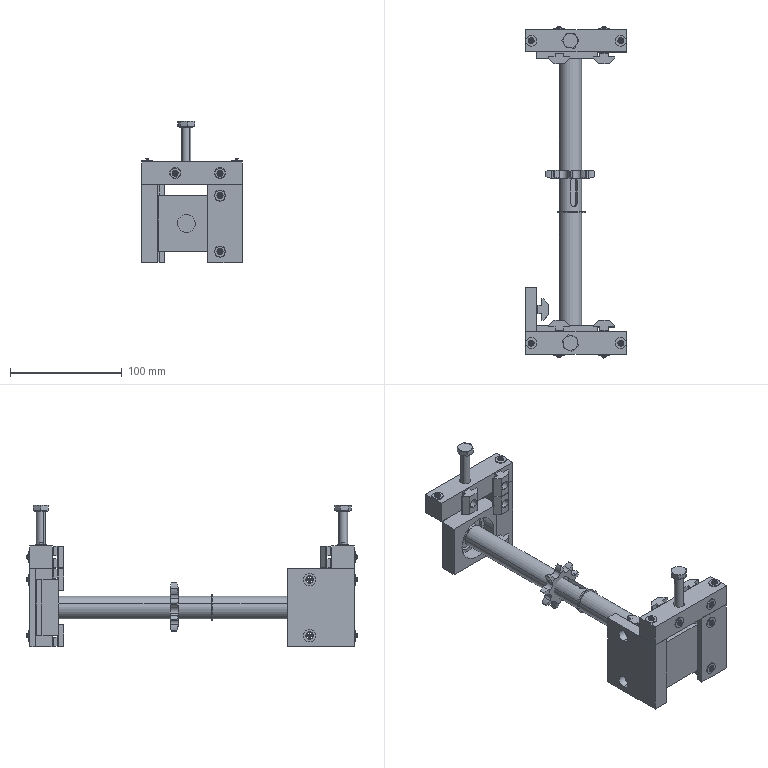Assembly | SolidWorks | mm | 63 component files | 63 solids | 1262 faces | box 90 x 296.4 x 126.4 mm | volume 353563 mm3 | plane 541 | cylinder 367 | torus 158 | sphere 100 | cone 96 | commonest cylinder face diameters 3 x64 4.2 x36 10 x28 1.6 x28 5.5 x24 6 x23 8 x20 22.466 x19
Bill of materials:
CTM-T-12-AG-02 | 2 | Q235A | Long rectangular bar with three through holes in the top face (a larger one near the middle and a smaller one near each end) and two cross holes through one long side face.
CTM-T-12-AG-03 | 1 | Q235A | Thick rectangular plate with an L-shaped profile: a small step or lip runs along one edge. Two through holes pass through the large face, and one hole is drilled into the narrow top end face.
CTM-T-12-AG-04 | 2 | Q235A | Solid rectangular block with a stepped (tongue-like) profile: a narrower raised section projects from one face, and a small notch shows at one top corner in isometric. No holes visible.
CTM-T-12-AG-05 | 2 | Q235A | Upright rectangular block with a rectangular notch (rabbet) at one top corner. Two through holes pass through one side face, and a single hole is drilled into the top face.
CTM-T-12-D-GD-03 | 1 | 45 | Stepped cylindrical shaft or pin: reduced-diameter journals at both ends and a slot (keyway-like) on the central section. Several circumferential seam lines divide the body into segments.
hex head bolts-full thread grade c gb | 2 |  | Hex-head bolt shape: chamfered hexagonal head on a plain cylindrical shank with a chamfered tip.
hexagon socket head cap screws gb | 14 |  | Socket-head cap screw shape: cylindrical head with a hexagonal socket recess, a plain cylindrical shank, and a chamfered end.
plain washers--product grade c gb | 12 |  | Plain flat washer: a thin annular disc with a central round hole.
self-aligning ball bearings gb | 2 |  | Ball-bearing-like assembly: an outer ring and an inner ring with a single row of 12 visible spherical rolling elements between them. No cage or shields visible.
ShaftRetainingRingTypeA-20-GB894.1-1986 | 2 | 65Mn | Flat split retaining ring (circlip shape) with a gap and two lugs, each with a small hole, beside the opening.
short pitch roller chain wheel_s_iso | 1 |  | Toothed disc with 9 teeth, rounded tooth gaps, and a plain central round bore; resembles a small chain sprocket.
spring lock washers--normal type gb | 12 |  | Split ring with a rectangular cross-section and one angled cut through the ring; resembles a split lock washer.
SquareNutBlock-MC6-8-30 | 2 | Purchased Part | Prismatic block with a constant T-shaped cross-section: a narrow rectangular stem on one side of a wider head whose outer edges are chamfered at about 45 degrees. One round through-hole runs through the wide flat face, roughly centred.
SquareNutBlock-MC8-8-40 | 8 | Purchased Part | Prismatic block with a T-shaped cross-section: a rectangular stem under a wider head with chamfered sides. A large round through-hole runs through the square face. A narrow rectangular slot is cut across the stem, partway into its depth, and meets the hole.
Mates:
1. concentric | self-aligning ball bearings gb-2 face at (40.4, -17, 35) dir (0, 1, 0) r 3 | CTM-T-12-D-GD-03-1 face at (40.4, -7, 35) dir (0, -1, 0) r 8.5
2. concentric | CTM-T-12-D-GD-03-1 face at (40.4, -270, 35) dir (0, 1, 0) r 10 | short pitch roller chain wheel_s_iso-1 face at (40.4, -123.269, 35) dir (0, -1, 0) r 6
3. width | self-aligning ball bearings gb-2 face at (43.023, -20, 36.455) dir (0, -1, 0) | self-aligning ball bearings gb-1 face at (43.75, -270, 38.933) dir (0, 1, 0) | CTM-T-12-D-GD-03-1 face at (40.4, -270, 35) dir (0, -1, 0) | CTM-T-12-D-GD-03-1 face at (40.4, -20, 35) dir (0, 1, 0)
4. width | CTM-T-12-AG-03-2 face at (0.4, -230, 0) dir (0, 0, -1) | CTM-T-12-AG-03-2 face at (0.4, -230, 70) dir (0, 0, 1) | CTM-T-12-AG-04-1 face at (15.4, -284, 60) dir (0, 0, 1) | CTM-T-12-AG-04-1 face at (15.4, -284, 10) dir (0, 0, -1)
5. concentric | self-aligning ball bearings gb-1 face at (40.4, -273, 35) dir (0, 1, 0) r 9.5 | CTM-T-12-AG-04-1 face at (40.4, -276, 35) dir (0, 1, 0) r 20
6. coincident | self-aligning ball bearings gb-1 face at (46.56, -276, 42.232) dir (0, -1, 0) | CTM-T-12-AG-04-1 face at (40.4, -276, 35) dir (0, 1, 0)
7. concentric | self-aligning ball bearings gb-2 face at (40.4, -17, 35) dir (0, 1, 0) r 9.5 | CTM-T-12-AG-04-2 face at (40.4, -14, 35) dir (0, -1, 0) r 20
8. coincident | self-aligning ball bearings gb-2 face at (46.808, -14, 38.554) dir (0, 1, 0) | CTM-T-12-AG-04-2 face at (40.4, -14, 35) dir (0, -1, 0)
9. coincident | CTM-T-12-AG-05-1 face at (59.4, 0, 70) dir (0, 0, 1) | CTM-T-12-AG-02-1 face at (90.4, 0, 70) dir (0, 0, -1)
10. coincident | CTM-T-12-AG-05-2 face at (59.4, -290, 70) dir (0, 0, 1) | CTM-T-12-AG-02-2 face at (90.4, -290, 70) dir (0, 0, -1)
11. distance | CTM-T-12-AG-02-2 face at (90.4, -270, 90) dir (0, 1, 0) | CTM-T-12-AG-02-1 face at (90.4, -20, 70) dir (0, -1, 0)
12. coincident | CTM-T-12-AG-02-2 face at (90.4, -290, 90) dir (0, 0, 1) | CTM-T-12-AG-02-1 face at (90.4, 0, 90) dir (0, 0, 1)
13. coincident | CTM-T-12-AG-02-2 face at (90.4, -270, 90) dir (1, 0, 0) | CTM-T-12-AG-02-1 face at (90.4, -20, 70) dir (1, 0, 0)
14. concentric | CTM-T-12-AG-02-2 face at (85.4, -280, 70) dir (0, 0, -1) r 3.5 | CTM-T-12-AG-05-2 face at (85.4, -280, 70) dir (0, 0, 1) r 3
15. concentric | CTM-T-12-AG-02-1 face at (85.4, -10, 90) dir (0, 0, 1) r 3.5 | CTM-T-12-AG-05-1 face at (85.4, -10, 70) dir (0, 0, 1) r 3
16. concentric | CTM-T-12-AG-02-2 face at (5.4, -280, 70) dir (0, 0, -1) r 3.5 | CTM-T-12-AG-03-2 face at (5.4, -280, 70) dir (0, 0, 1) r 3
17. coincident | CTM-T-12-AG-02-2 face at (90.4, -290, 90) dir (0, -1, 0) | CTM-T-12-AG-05-2 face at (90.4, -290, 70) dir (0, -1, 0)
18. coincident | CTM-T-12-AG-02-2 face at (90.4, -290, 90) dir (0, -1, 0) | CTM-T-12-AG-03-2 face at (0.4, -290, 0) dir (0, -1, 0)
19. width | CTM-T-12-AG-04-2 face at (59.4, -6, 10) dir (0, 1, 0) | CTM-T-12-AG-04-1 face at (59.4, -284, 60) dir (0, -1, 0) | CTM-T-12-AG-05-1 face at (59.4, -5, 0) dir (0, -1, 0) | CTM-T-12-AG-05-2 face at (59.4, -285, 70) dir (0, 1, 0)
20. coincident | CTM-T-12-D-GD-03-1 face at (45.383, -155, 40.14) dir (-0.9436, 0, 0.3311) | short pitch roller chain wheel_s_iso-1 face at (43.231, -106.669, 34.007) dir (-0.9436, 0, 0.3311)
21. coincident | CTM-T-12-D-GD-03-1 face at (40.4, -270, 35) dir (0, -1, 0) | self-aligning ball bearings gb-1 face at (43.75, -270, 38.933) dir (0, 1, 0)
22. coincident | CTM-T-12-AG-04-1 face at (59.4, -279, 60) dir (1, 0, 0) | CTM-T-12-AG-05-2 face at (59.4, -290, 70) dir (-1, 0, 0)
23. coincident | CTM-T-12-AG-04-2 face at (59.4, -11, 10) dir (1, 0, 0) | CTM-T-12-AG-05-1 face at (59.4, 0, 0) dir (-1, 0, 0)
24. concentric | CTM-T-12-D-GD-03-1 face at (40.4, -270, 35) dir (0, 1, 0) r 10 | ShaftRetainingRingTypeA-20-GB894.1-1986-1 face at (40.4, -127.35, 35) dir (0, 1, 0) r 11.25
25. concentric | CTM-T-12-D-GD-03-1 face at (40.4, -270, 35) dir (0, 1, 0) r 10 | ShaftRetainingRingTypeA-20-GB894.1-1986-2 face at (40.4, -163.65, 35) dir (0, 1, 0) r 11.25
26. coincident | CTM-T-12-D-GD-03-1 face at (40.4, -163.65, 35) dir (0, 1, 0) | ShaftRetainingRingTypeA-20-GB894.1-1986-2 face at (46.83, -163.65, 24.573) dir (0, -1, 0)
27. coincident | CTM-T-12-D-GD-03-1 face at (40.4, -126.35, 35) dir (0, -1, 0) | ShaftRetainingRingTypeA-20-GB894.1-1986-1 face at (46.83, -126.35, 24.573) dir (0, 1, 0)
28. concentric | hexagon socket head cap screws gb-1 face at (85.4, -10, 85.6) dir (0, 0, 1) r 0.8 | plain washers--product grade c gb-3 face at (85.4, -10, 90) dir (0, 0, 1) r 2.75
29. coincident | CTM-T-12-AG-02-1 face at (90.4, 0, 90) dir (0, 0, 1) | plain washers--product grade c gb-3 face at (85.4, -10, 90) dir (0, 0, -1)
30. concentric | hexagon socket head cap screws gb-1 face at (85.4, -10, 85.6) dir (0, 0, 1) r 0.8 | spring lock washers--normal type gb-1 face at (85.4, -10, 91) dir (0, 0, 1) r 1.5
31. coincident | plain washers--product grade c gb-3 face at (85.4, -10, 91) dir (0, 0, 1) | spring lock washers--normal type gb-1 face at (85.4, -10, 91) dir (0, 0, -1)
32. concentric | CTM-T-12-AG-02-1 face at (85.4, -10, 90) dir (0, 0, 1) r 3.5 | hexagon socket head cap screws gb-1 face at (85.4, -10, 85.6) dir (0, 0, 1) r 0.8
33. coincident | hexagon socket head cap screws gb-1 face at (85.4, -10, 91.6) dir (0, 0, -1) | spring lock washers--normal type gb-1 face at (85.4, -10, 91.6) dir (0, 0, 1)
34. concentric | hexagon socket head cap screws gb-2 face at (5.4, -10, 85.6) dir (0, 0, 1) r 0.8 | plain washers--product grade c gb-4 face at (5.4, -10, 90) dir (0, 0, 1) r 2.75
35. coincident | CTM-T-12-AG-02-1 face at (90.4, 0, 90) dir (0, 0, 1) | plain washers--product grade c gb-4 face at (5.4, -10, 90) dir (0, 0, -1)
36. concentric | hexagon socket head cap screws gb-2 face at (5.4, -10, 85.6) dir (0, 0, 1) r 0.8 | spring lock washers--normal type gb-2 face at (5.4, -10, 91) dir (0, 0, 1) r 1.5
37. coincident | plain washers--product grade c gb-4 face at (5.4, -10, 91) dir (0, 0, 1) | spring lock washers--normal type gb-2 face at (5.4, -10, 91) dir (0, 0, -1)
38. concentric | CTM-T-12-AG-02-1 face at (5.4, -10, 90) dir (0, 0, 1) r 3.5 | hexagon socket head cap screws gb-2 face at (5.4, -10, 85.6) dir (0, 0, 1) r 0.8
39. coincident | hexagon socket head cap screws gb-2 face at (5.4, -10, 91.6) dir (0, 0, -1) | spring lock washers--normal type gb-2 face at (5.4, -10, 91.6) dir (0, 0, 1)
40. concentric | hexagon socket head cap screws gb-3 face at (85.4, -280, 85.6) dir (0, 0, 1) r 0.8 | plain washers--product grade c gb-7 face at (85.4, -280, 90) dir (0, 0, 1) r 2.75
41. coincident | CTM-T-12-AG-02-2 face at (90.4, -290, 90) dir (0, 0, 1) | plain washers--product grade c gb-7 face at (85.4, -280, 90) dir (0, 0, -1)
42. concentric | hexagon socket head cap screws gb-3 face at (85.4, -280, 85.6) dir (0, 0, 1) r 0.8 | spring lock washers--normal type gb-3 face at (85.4, -280, 91) dir (0, 0, 1) r 1.5
43. coincident | plain washers--product grade c gb-7 face at (85.4, -280, 91) dir (0, 0, 1) | spring lock washers--normal type gb-3 face at (85.4, -280, 91) dir (0, 0, -1)
44. concentric | CTM-T-12-AG-02-2 face at (85.4, -280, 70) dir (0, 0, -1) r 3.5 | hexagon socket head cap screws gb-3 face at (85.4, -280, 85.6) dir (0, 0, 1) r 0.8
45. coincident | hexagon socket head cap screws gb-3 face at (85.4, -280, 91.6) dir (0, 0, -1) | spring lock washers--normal type gb-3 face at (85.4, -280, 91.6) dir (0, 0, 1)
46. concentric | hexagon socket head cap screws gb-4 face at (5.4, -280, 85.6) dir (0, 0, 1) r 0.8 | plain washers--product grade c gb-8 face at (5.4, -280, 90) dir (0, 0, 1) r 2.75
47. coincident | CTM-T-12-AG-02-2 face at (90.4, -290, 90) dir (0, 0, 1) | plain washers--product grade c gb-8 face at (5.4, -280, 90) dir (0, 0, -1)
48. concentric | hexagon socket head cap screws gb-4 face at (5.4, -280, 85.6) dir (0, 0, 1) r 0.8 | spring lock washers--normal type gb-4 face at (5.4, -280, 91) dir (0, 0, 1) r 1.5
49. coincident | plain washers--product grade c gb-8 face at (5.4, -280, 91) dir (0, 0, 1) | spring lock washers--normal type gb-4 face at (5.4, -280, 91) dir (0, 0, -1)
50. concentric | CTM-T-12-AG-02-2 face at (5.4, -280, 70) dir (0, 0, -1) r 3.5 | hexagon socket head cap screws gb-4 face at (5.4, -280, 85.6) dir (0, 0, 1) r 0.8
51. coincident | hexagon socket head cap screws gb-4 face at (5.4, -280, 91.6) dir (0, 0, -1) | spring lock washers--normal type gb-4 face at (5.4, -280, 91.6) dir (0, 0, 1)
52. concentric | hexagon socket head cap screws gb-5 face at (70.4, -4.4, 60) dir (0, 1, 0) r 0.8 | plain washers--product grade c gb-11 face at (70.4, 0, 60) dir (0, 1, 0) r 2.75
53. coincident | CTM-T-12-AG-05-1 face at (90.4, 0, 0) dir (0, 1, 0) | plain washers--product grade c gb-11 face at (70.4, 0, 60) dir (0, -1, 0)
54. concentric | hexagon socket head cap screws gb-5 face at (70.4, -4.4, 60) dir (0, 1, 0) r 0.8 | spring lock washers--normal type gb-5 face at (70.4, 1, 60) dir (0, 1, 0) r 1.5
55. coincident | plain washers--product grade c gb-11 face at (70.4, 1, 60) dir (0, 1, 0) | spring lock washers--normal type gb-5 face at (70.4, 1, 60) dir (0, -1, 0)
56. concentric | CTM-T-12-AG-05-1 face at (70.4, 0, 60) dir (0, 1, 0) r 4.5 | hexagon socket head cap screws gb-5 face at (70.4, -4.4, 60) dir (0, 1, 0) r 0.8
57. coincident | hexagon socket head cap screws gb-5 face at (70.4, 1.6, 60) dir (0, -1, 0) | spring lock washers--normal type gb-5 face at (70.4, 1.6, 60) dir (0, 1, 0)
58. concentric | hexagon socket head cap screws gb-6 face at (70.4, -4.4, 10) dir (0, 1, 0) r 0.8 | plain washers--product grade c gb-12 face at (70.4, 0, 10) dir (0, 1, 0) r 2.75
59. coincident | CTM-T-12-AG-05-1 face at (90.4, 0, 0) dir (0, 1, 0) | plain washers--product grade c gb-12 face at (70.4, 0, 10) dir (0, -1, 0)
60. concentric | hexagon socket head cap screws gb-6 face at (70.4, -4.4, 10) dir (0, 1, 0) r 0.8 | spring lock washers--normal type gb-6 face at (70.4, 1, 10) dir (0, 1, 0) r 1.5
61. coincident | plain washers--product grade c gb-12 face at (70.4, 1, 10) dir (0, 1, 0) | spring lock washers--normal type gb-6 face at (70.4, 1, 10) dir (0, -1, 0)
62. concentric | CTM-T-12-AG-05-1 face at (70.4, 0, 10) dir (0, 1, 0) r 4.5 | hexagon socket head cap screws gb-6 face at (70.4, -4.4, 10) dir (0, 1, 0) r 0.8
63. coincident | hexagon socket head cap screws gb-6 face at (70.4, 1.6, 10) dir (0, -1, 0) | spring lock washers--normal type gb-6 face at (70.4, 1.6, 10) dir (0, 1, 0)
64. concentric | hexagon socket head cap screws gb-7 face at (70.4, -285.6, 10) dir (0, -1, 0) r 0.8 | plain washers--product grade c gb-17 face at (70.4, -290, 10) dir (0, -1, 0) r 2.75
65. coincident | CTM-T-12-AG-05-2 face at (90.4, -290, 70) dir (0, -1, 0) | plain washers--product grade c gb-17 face at (70.4, -290, 10) dir (0, 1, 0)
66. concentric | hexagon socket head cap screws gb-7 face at (70.4, -285.6, 10) dir (0, -1, 0) r 0.8 | spring lock washers--normal type gb-11 face at (70.4, -291, 10) dir (0, -1, 0) r 1.5
67. coincident | plain washers--product grade c gb-17 face at (70.4, -291, 10) dir (0, -1, 0) | spring lock washers--normal type gb-11 face at (70.4, -291, 10) dir (0, 1, 0)
68. concentric | CTM-T-12-AG-05-2 face at (70.4, -290, 10) dir (0, -1, 0) r 4.5 | hexagon socket head cap screws gb-7 face at (70.4, -285.6, 10) dir (0, -1, 0) r 0.8
69. coincident | hexagon socket head cap screws gb-7 face at (70.4, -291.6, 10) dir (0, 1, 0) | spring lock washers--normal type gb-11 face at (70.4, -291.6, 10) dir (0, -1, 0)
70. concentric | hexagon socket head cap screws gb-8 face at (70.4, -285.6, 60) dir (0, -1, 0) r 0.8 | plain washers--product grade c gb-18 face at (70.4, -290, 60) dir (0, -1, 0) r 2.75
71. coincident | CTM-T-12-AG-05-2 face at (90.4, -290, 70) dir (0, -1, 0) | plain washers--product grade c gb-18 face at (70.4, -290, 60) dir (0, 1, 0)
72. concentric | hexagon socket head cap screws gb-8 face at (70.4, -285.6, 60) dir (0, -1, 0) r 0.8 | spring lock washers--normal type gb-12 face at (70.4, -291, 60) dir (0, -1, 0) r 1.5
73. coincident | plain washers--product grade c gb-18 face at (70.4, -291, 60) dir (0, -1, 0) | spring lock washers--normal type gb-12 face at (70.4, -291, 60) dir (0, 1, 0)
74. concentric | CTM-T-12-AG-05-2 face at (70.4, -290, 60) dir (0, -1, 0) r 4.5 | hexagon socket head cap screws gb-8 face at (70.4, -285.6, 60) dir (0, -1, 0) r 0.8
75. coincident | hexagon socket head cap screws gb-8 face at (70.4, -291.6, 60) dir (0, 1, 0) | spring lock washers--normal type gb-12 face at (70.4, -291.6, 60) dir (0, -1, 0)
76. concentric | CTM-T-12-AG-03-2 face at (0.4, -250, 60) dir (-1, 0, 0) r 3.3 | hexagon socket head cap screws gb-18 face at (13.2, -250, 60) dir (-1, 0, 0) r 0.8
77. coincident | CTM-T-12-AG-03-2 face at (7.2, -253.3, 60) dir (-1, 0, 0) | hexagon socket head cap screws gb-18 face at (7.2, -250, 60) dir (1, 0, 0)
78. concentric | CTM-T-12-AG-03-2 face at (0.4, -250, 10) dir (-1, 0, 0) r 3.3 | hexagon socket head cap screws gb-19 face at (13.2, -250, 10) dir (-1, 0, 0) r 0.8
79. coincident | CTM-T-12-AG-03-2 face at (7.2, -253.3, 10) dir (-1, 0, 0) | hexagon socket head cap screws gb-19 face at (7.2, -250, 10) dir (1, 0, 0)
80. concentric | SquareNutBlock-MC8-8-40-1 face at (70.4, -259.6, 60) dir (0, 1, 0) r 4 | hexagon socket head cap screws gb-8 face at (70.4, -285.6, 60) dir (0, -1, 0) r 0.8
81. parallel | CTM-T-12-AG-05-2 face at (90.4, -290, 70) dir (1, 0, 0) | SquareNutBlock-MC8-8-40-1 face at (79.9, -264.4, 69.65) dir (1, 0, 0)
82. distance | SquareNutBlock-MC8-8-40-1 face at (74.15, -269, 69.65) dir (0, -1, 0) | CTM-T-12-AG-05-2 face at (90.4, -270, 70) dir (0, 1, 0)
83. parallel | CTM-T-12-AG-05-2 face at (90.4, -290, 70) dir (1, 0, 0) | SquareNutBlock-MC8-8-40-2 face at (79.9, -264.4, 19.65) dir (1, 0, 0)
84. distance | SquareNutBlock-MC8-8-40-2 face at (74.15, -269, 19.65) dir (0, -1, 0) | CTM-T-12-AG-05-2 face at (90.4, -270, 70) dir (0, 1, 0)
85. concentric | SquareNutBlock-MC8-8-40-2 face at (70.4, -259.6, 10) dir (0, 1, 0) r 4 | hexagon socket head cap screws gb-7 face at (70.4, -285.6, 10) dir (0, -1, 0) r 0.8
86. concentric | SquareNutBlock-MC8-8-40-3 face at (70.4, -30.4, 60) dir (0, -1, 0) r 4 | hexagon socket head cap screws gb-5 face at (70.4, -4.4, 60) dir (0, 1, 0) r 0.8
87. parallel | CTM-T-12-AG-05-1 face at (90.4, 0, 0) dir (1, 0, 0) | SquareNutBlock-MC8-8-40-3 face at (79.9, -25.6, 50.35) dir (1, 0, 0)
88. distance | SquareNutBlock-MC8-8-40-3 face at (74.15, -21, 50.35) dir (0, 1, 0) | CTM-T-12-AG-05-1 face at (90.4, -20, 0) dir (0, -1, 0)
89. parallel | CTM-T-12-AG-05-1 face at (90.4, 0, 0) dir (1, 0, 0) | SquareNutBlock-MC8-8-40-4 face at (79.9, -25.6, 0.35) dir (1, 0, 0)
90. distance | SquareNutBlock-MC8-8-40-4 face at (74.15, -21, 0.35) dir (0, 1, 0) | CTM-T-12-AG-05-1 face at (90.4, -20, 0) dir (0, -1, 0)
91. concentric | SquareNutBlock-MC8-8-40-4 face at (70.4, -30.4, 10) dir (0, -1, 0) r 4 | hexagon socket head cap screws gb-6 face at (70.4, -4.4, 10) dir (0, 1, 0) r 0.8
92. concentric | SquareNutBlock-MC6-8-30-1 face at (20.8, -250, 10) dir (1, 0, 0) r 3 | hexagon socket head cap screws gb-19 face at (13.2, -250, 10) dir (-1, 0, 0) r 0.8
93. parallel | CTM-T-12-AG-03-2 face at (0.4, -230, 0) dir (0, 1, 0) | SquareNutBlock-MC6-8-30-1 face at (14.9, -240.5, 19.65) dir (0, 1, 0)
94. distance | SquareNutBlock-MC6-8-30-1 face at (11.4, -253.75, 19.65) dir (-1, 0, 0) | CTM-T-12-AG-03-2 face at (10.4, -285, 0) dir (1, 0, 0)
95. parallel | CTM-T-12-AG-03-2 face at (0.4, -230, 0) dir (0, 1, 0) | SquareNutBlock-MC6-8-30-2 face at (14.9, -240.5, 69.65) dir (0, 1, 0)
96. distance | SquareNutBlock-MC6-8-30-2 face at (11.4, -253.75, 69.65) dir (-1, 0, 0) | CTM-T-12-AG-03-2 face at (10.4, -285, 0) dir (1, 0, 0)
97. concentric | SquareNutBlock-MC6-8-30-2 face at (20.8, -250, 60) dir (1, 0, 0) r 3 | hexagon socket head cap screws gb-18 face at (13.2, -250, 60) dir (-1, 0, 0) r 0.8
98. concentric | hexagon socket head cap screws gb-14 face at (30.4, -285.6, 80) dir (0, -1, 0) r 0.8 | plain washers--product grade c gb-22 face at (30.4, -290, 80) dir (0, -1, 0) r 2.75
99. coincident | CTM-T-12-AG-02-2 face at (90.4, -290, 90) dir (0, -1, 0) | plain washers--product grade c gb-22 face at (30.4, -290, 80) dir (0, 1, 0)
100. concentric | hexagon socket head cap screws gb-14 face at (30.4, -285.6, 80) dir (0, -1, 0) r 0.8 | spring lock washers--normal type gb-14 face at (30.4, -291, 80) dir (0, -1, 0) r 1.5
101. coincident | plain washers--product grade c gb-22 face at (30.4, -291, 80) dir (0, -1, 0) | spring lock washers--normal type gb-14 face at (30.4, -291, 80) dir (0, 1, 0)
102. concentric | CTM-T-12-AG-02-2 face at (30.4, -270, 80) dir (0, 1, 0) r 4.5 | hexagon socket head cap screws gb-14 face at (30.4, -285.6, 80) dir (0, -1, 0) r 0.8
103. coincident | hexagon socket head cap screws gb-14 face at (30.4, -291.6, 80) dir (0, 1, 0) | spring lock washers--normal type gb-14 face at (30.4, -291.6, 80) dir (0, -1, 0)
104. concentric | hexagon socket head cap screws gb-15 face at (70.4, -285.6, 80) dir (0, -1, 0) r 0.8 | plain washers--product grade c gb-23 face at (70.4, -290, 80) dir (0, -1, 0) r 2.75
105. coincident | CTM-T-12-AG-02-2 face at (90.4, -290, 90) dir (0, -1, 0) | plain washers--product grade c gb-23 face at (70.4, -290, 80) dir (0, 1, 0)
106. concentric | hexagon socket head cap screws gb-15 face at (70.4, -285.6, 80) dir (0, -1, 0) r 0.8 | spring lock washers--normal type gb-15 face at (70.4, -291, 80) dir (0, -1, 0) r 1.5
107. coincident | plain washers--product grade c gb-23 face at (70.4, -291, 80) dir (0, -1, 0) | spring lock washers--normal type gb-15 face at (70.4, -291, 80) dir (0, 1, 0)
108. concentric | CTM-T-12-AG-02-2 face at (70.4, -270, 80) dir (0, 1, 0) r 4.5 | hexagon socket head cap screws gb-15 face at (70.4, -285.6, 80) dir (0, -1, 0) r 0.8
109. coincident | hexagon socket head cap screws gb-15 face at (70.4, -291.6, 80) dir (0, 1, 0) | spring lock washers--normal type gb-15 face at (70.4, -291.6, 80) dir (0, -1, 0)
110. concentric | SquareNutBlock-MC8-8-40-7 face at (70.4, -259.6, 80) dir (0, 1, 0) r 4 | hexagon socket head cap screws gb-15 face at (70.4, -285.6, 80) dir (0, -1, 0) r 0.8
111. parallel | CTM-T-12-AG-02-2 face at (90.4, -270, 90) dir (1, 0, 0) | SquareNutBlock-MC8-8-40-7 face at (79.9, -264.4, 89.65) dir (1, 0, 0)
112. distance | SquareNutBlock-MC8-8-40-7 face at (74.15, -269, 89.65) dir (0, -1, 0) | CTM-T-12-AG-02-2 face at (90.4, -270, 90) dir (0, 1, 0)
113. parallel | CTM-T-12-AG-02-2 face at (90.4, -270, 90) dir (1, 0, 0) | SquareNutBlock-MC8-8-40-8 face at (39.9, -264.4, 89.65) dir (1, 0, 0)
114. distance | SquareNutBlock-MC8-8-40-8 face at (34.15, -269, 89.65) dir (0, -1, 0) | CTM-T-12-AG-02-2 face at (90.4, -270, 90) dir (0, 1, 0)
115. concentric | SquareNutBlock-MC8-8-40-8 face at (30.4, -259.6, 80) dir (0, 1, 0) r 4 | hexagon socket head cap screws gb-14 face at (30.4, -285.6, 80) dir (0, -1, 0) r 0.8
116. concentric | hexagon socket head cap screws gb-16 face at (30.4, -4.4, 80) dir (0, 1, 0) r 0.8 | plain washers--product grade c gb-26 face at (30.4, 0, 80) dir (0, 1, 0) r 2.75
117. coincident | CTM-T-12-AG-02-1 face at (90.4, 0, 70) dir (0, 1, 0) | plain washers--product grade c gb-26 face at (30.4, 0, 80) dir (0, -1, 0)
118. concentric | hexagon socket head cap screws gb-16 face at (30.4, -4.4, 80) dir (0, 1, 0) r 0.8 | spring lock washers--normal type gb-16 face at (30.4, 1, 80) dir (0, 1, 0) r 1.5
119. coincident | plain washers--product grade c gb-26 face at (30.4, 1, 80) dir (0, 1, 0) | spring lock washers--normal type gb-16 face at (30.4, 1, 80) dir (0, -1, 0)
120. concentric | CTM-T-12-AG-02-1 face at (30.4, -20, 80) dir (0, -1, 0) r 4.5 | hexagon socket head cap screws gb-16 face at (30.4, -4.4, 80) dir (0, 1, 0) r 0.8
121. coincident | hexagon socket head cap screws gb-16 face at (30.4, 1.6, 80) dir (0, -1, 0) | spring lock washers--normal type gb-16 face at (30.4, 1.6, 80) dir (0, 1, 0)
122. concentric | hexagon socket head cap screws gb-17 face at (70.4, -4.4, 80) dir (0, 1, 0) r 0.8 | plain washers--product grade c gb-27 face at (70.4, 0, 80) dir (0, 1, 0) r 2.75
123. coincident | CTM-T-12-AG-02-1 face at (90.4, 0, 70) dir (0, 1, 0) | plain washers--product grade c gb-27 face at (70.4, 0, 80) dir (0, -1, 0)
124. concentric | hexagon socket head cap screws gb-17 face at (70.4, -4.4, 80) dir (0, 1, 0) r 0.8 | spring lock washers--normal type gb-17 face at (70.4, 1, 80) dir (0, 1, 0) r 1.5
125. coincident | plain washers--product grade c gb-27 face at (70.4, 1, 80) dir (0, 1, 0) | spring lock washers--normal type gb-17 face at (70.4, 1, 80) dir (0, -1, 0)
126. concentric | CTM-T-12-AG-02-1 face at (70.4, -20, 80) dir (0, -1, 0) r 4.5 | hexagon socket head cap screws gb-17 face at (70.4, -4.4, 80) dir (0, 1, 0) r 0.8
127. coincident | hexagon socket head cap screws gb-17 face at (70.4, 1.6, 80) dir (0, -1, 0) | spring lock washers--normal type gb-17 face at (70.4, 1.6, 80) dir (0, 1, 0)
128. concentric | SquareNutBlock-MC8-8-40-9 face at (70.4, -30.4, 80) dir (0, -1, 0) r 4 | hexagon socket head cap screws gb-17 face at (70.4, -4.4, 80) dir (0, 1, 0) r 0.8
129. parallel | CTM-T-12-AG-02-1 face at (90.4, -20, 70) dir (1, 0, 0) | SquareNutBlock-MC8-8-40-9 face at (79.9, -25.6, 70.35) dir (1, 0, 0)
130. distance | SquareNutBlock-MC8-8-40-9 face at (74.15, -21, 70.35) dir (0, 1, 0) | CTM-T-12-AG-02-1 face at (90.4, -20, 70) dir (0, -1, 0)
131. parallel | CTM-T-12-AG-02-1 face at (90.4, -20, 70) dir (1, 0, 0) | SquareNutBlock-MC8-8-40-10 face at (39.9, -25.6, 70.35) dir (1, 0, 0)
132. distance | SquareNutBlock-MC8-8-40-10 face at (34.15, -21, 70.35) dir (0, 1, 0) | CTM-T-12-AG-02-1 face at (90.4, -20, 70) dir (0, -1, 0)
133. concentric | SquareNutBlock-MC8-8-40-10 face at (30.4, -30.4, 80) dir (0, -1, 0) r 4 | hexagon socket head cap screws gb-16 face at (30.4, -4.4, 80) dir (0, 1, 0) r 0.8
134. concentric | CTM-T-12-AG-02-1 face at (40.4, -10, 90) dir (0, 0, 1) r 5 | hex head bolts-full thread grade c gb-1 face at (40.4, -10, 86.1) dir (0, 0, 1) r 4
135. concentric | hexagon nuts grade c gb-1 face at (40.4, -10, 90) dir (0, 0, 1) r 4.188 | hex head bolts-full thread grade c gb-1 face at (40.4, -10, 86.1) dir (0, 0, 1) r 4
136. coincident | CTM-T-12-AG-02-1 face at (90.4, 0, 90) dir (0, 0, 1) | hexagon nuts grade c gb-1 face at (42.071, -19.085, 90) dir (0, 0, -1)
137. concentric | hexagon nuts grade c gb-3 face at (40.4, -280, 90) dir (0, 0, 1) r 4.188 | hex head bolts-full thread grade c gb-3 face at (40.4, -280, 86.1) dir (0, 0, 1) r 4
138. concentric | CTM-T-12-AG-02-2 face at (40.4, -280, 70) dir (0, 0, -1) r 5 | hex head bolts-full thread grade c gb-3 face at (40.4, -280, 86.1) dir (0, 0, 1) r 4
139. coincident | CTM-T-12-AG-02-2 face at (90.4, -290, 90) dir (0, 0, 1) | hexagon nuts grade c gb-3 face at (38.729, -270.915, 90) dir (0, 0, -1)